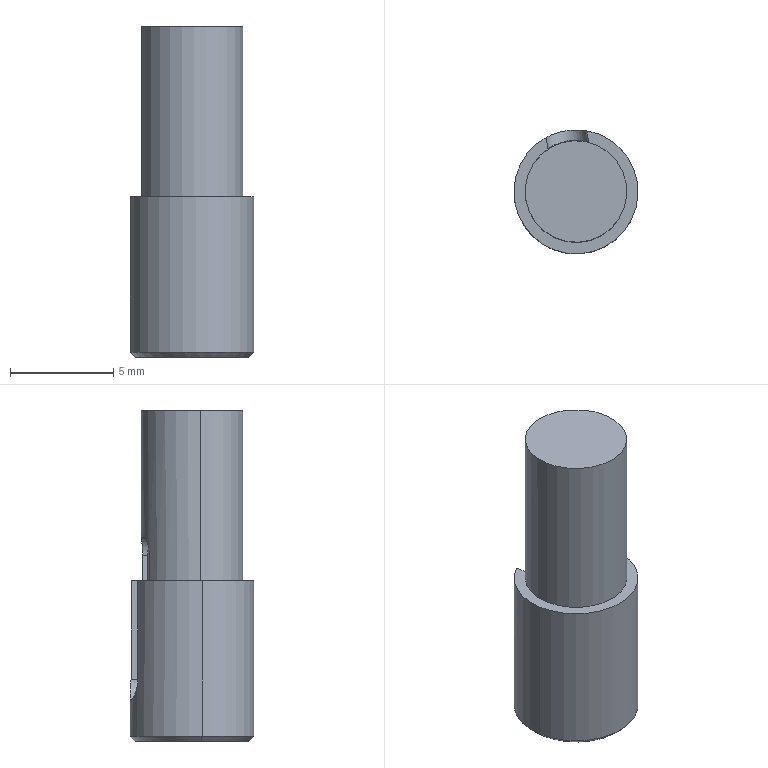Component | SolidWorks | GMotorAxis-1 | 1 solid | 18 faces | box 6 x 6 x 16 mm | volume 268 mm3 | cylinder 9 | plane 7 | cone 2 | commonest cylinder face diameters 2 x3 4.917 x2 5 x2 6 x2
STEP:
#1=COLOUR_RGB('',0.7922,0.8196,0.9333);
#2=FILL_AREA_STYLE_COLOUR('',#1);
#3=FILL_AREA_STYLE('',(#2));
#4=SURFACE_STYLE_FILL_AREA(#3);
#5=SURFACE_SIDE_STYLE('',(#4));
#6=SURFACE_STYLE_USAGE(.BOTH.,#5);
#7=PRESENTATION_STYLE_ASSIGNMENT((#6));
#8=CARTESIAN_POINT('',(-0.6803,0.01391,0.7392));
#9=VERTEX_POINT('',#8);
#10=CARTESIAN_POINT('',(-0.7226,-0.08267,0.7392));
#11=VERTEX_POINT('',#10);
#12=CARTESIAN_POINT('',(-0.6271,-0.06694,0.7392));
#13=DIRECTION('',(0.,0.,1.));
#14=DIRECTION('',(0.9867,0.1625,0.));
#15=AXIS2_PLACEMENT_3D('',#12,#13,#14);
#16=CIRCLE('',#15,0.09679);
#17=EDGE_CURVE('',#9,#11,#16,.T.);
#18=ORIENTED_EDGE('',*,*,#17,.T.);
#19=CARTESIAN_POINT('',(-0.7226,-0.08267,1.063));
#20=VERTEX_POINT('',#19);
#21=CARTESIAN_POINT('',(-0.7226,-0.08267,0.7392));
#22=DIRECTION('',(0.,0.,1.));
#23=VECTOR('',#22,39.37);
#24=LINE('',#21,#23);
#25=EDGE_CURVE('',#11,#20,#24,.T.);
#26=ORIENTED_EDGE('',*,*,#25,.T.);
#27=CARTESIAN_POINT('',(-0.5316,-0.0512,1.063));
#28=VERTEX_POINT('',#27);
#29=CARTESIAN_POINT('',(-0.6271,-0.06694,1.063));
#30=DIRECTION('',(0.,0.,1.));
#31=DIRECTION('',(0.9867,0.1625,0.));
#32=AXIS2_PLACEMENT_3D('',#29,#30,#31);
#33=CIRCLE('',#32,0.09679);
#34=EDGE_CURVE('',#28,#20,#33,.T.);
#35=ORIENTED_EDGE('',*,*,#34,.F.);
#36=CARTESIAN_POINT('',(-0.5316,-0.0512,0.7392));
#37=VERTEX_POINT('',#36);
#38=CARTESIAN_POINT('',(-0.5316,-0.0512,0.7392));
#39=DIRECTION('',(0.,0.,1.));
#40=VECTOR('',#39,39.37);
#41=LINE('',#38,#40);
#42=EDGE_CURVE('',#37,#28,#41,.T.);
#43=ORIENTED_EDGE('',*,*,#42,.F.);
#44=CARTESIAN_POINT('',(-0.6026,0.02671,0.7392));
#45=VERTEX_POINT('',#44);
#46=CARTESIAN_POINT('',(-0.6271,-0.06694,0.7392));
#47=DIRECTION('',(0.,0.,1.));
#48=DIRECTION('',(0.9867,0.1625,0.));
#49=AXIS2_PLACEMENT_3D('',#46,#47,#48);
#50=CIRCLE('',#49,0.09679);
#51=EDGE_CURVE('',#37,#45,#50,.T.);
#52=ORIENTED_EDGE('',*,*,#51,.T.);
#53=CARTESIAN_POINT('',(-0.6026,0.02671,0.7874));
#54=VERTEX_POINT('',#53);
#55=CARTESIAN_POINT('',(-0.6026,0.02671,0.7392));
#56=DIRECTION('',(0.,0.,1.));
#57=VECTOR('',#56,39.37);
#58=LINE('',#55,#57);
#59=EDGE_CURVE('',#45,#54,#58,.T.);
#60=ORIENTED_EDGE('',*,*,#59,.T.);
#61=CARTESIAN_POINT('',(-0.6428,0.02857,0.8268));
#62=VERTEX_POINT('',#61);
#63=CARTESIAN_POINT('',(-0.6026,0.02671,0.7874));
#64=CARTESIAN_POINT('',(-0.6026,0.02671,0.7927));
#65=CARTESIAN_POINT('',(-0.6037,0.02702,0.7978));
#66=CARTESIAN_POINT('',(-0.6079,0.02796,0.8073));
#67=CARTESIAN_POINT('',(-0.611,0.02858,0.8117));
#68=CARTESIAN_POINT('',(-0.6184,0.02954,0.8188));
#69=CARTESIAN_POINT('',(-0.6229,0.02988,0.8218));
#70=CARTESIAN_POINT('',(-0.6325,0.02982,0.8257));
#71=CARTESIAN_POINT('',(-0.6377,0.02941,0.8268));
#72=CARTESIAN_POINT('',(-0.6428,0.02857,0.8268));
#73=B_SPLINE_CURVE_WITH_KNOTS('',3,(#63,#64,#65,#66,#67,#68,#69,#70,#71,#72),.UNSPECIFIED.,.F.,.F.,(4,2,2,2,4),(0.,0.0003952,0.0007905,0.001186,0.001581),.UNSPECIFIED.);
#74=EDGE_CURVE('',#54,#62,#73,.T.);
#75=ORIENTED_EDGE('',*,*,#74,.T.);
#76=CARTESIAN_POINT('',(-0.6803,0.01391,0.7874));
#77=VERTEX_POINT('',#76);
#78=CARTESIAN_POINT('',(-0.6428,0.02857,0.8268));
#79=CARTESIAN_POINT('',(-0.6479,0.02772,0.8268));
#80=CARTESIAN_POINT('',(-0.653,0.02645,0.8257));
#81=CARTESIAN_POINT('',(-0.6622,0.02339,0.8217));
#82=CARTESIAN_POINT('',(-0.6663,0.02165,0.8188));
#83=CARTESIAN_POINT('',(-0.673,0.01835,0.8116));
#84=CARTESIAN_POINT('',(-0.6757,0.01679,0.8073));
#85=CARTESIAN_POINT('',(-0.6793,0.01457,0.7979));
#86=CARTESIAN_POINT('',(-0.6803,0.01391,0.7927));
#87=CARTESIAN_POINT('',(-0.6803,0.01391,0.7874));
#88=B_SPLINE_CURVE_WITH_KNOTS('',3,(#78,#79,#80,#81,#82,#83,#84,#85,#86,#87),.UNSPECIFIED.,.F.,.F.,(4,2,2,2,4),(0.001581,0.001976,0.00237,0.002765,0.003159),.UNSPECIFIED.);
#89=EDGE_CURVE('',#62,#77,#88,.T.);
#90=ORIENTED_EDGE('',*,*,#89,.T.);
#91=CARTESIAN_POINT('',(-0.6803,0.01391,0.7392));
#92=DIRECTION('',(0.,0.,-1.));
#93=VECTOR('',#92,39.37);
#94=LINE('',#91,#93);
#95=EDGE_CURVE('',#77,#9,#94,.T.);
#96=ORIENTED_EDGE('',*,*,#95,.T.);
#97=EDGE_LOOP('',(#18,#26,#35,#43,#52,#60,#75,#90,#96));
#98=FACE_OUTER_BOUND('',#97,.T.);
#99=CARTESIAN_POINT('',(-0.6271,-0.06694,0.7392));
#100=DIRECTION('',(0.,0.,1.));
#101=DIRECTION('',(0.9867,0.1625,0.));
#102=AXIS2_PLACEMENT_3D('',#99,#100,#101);
#103=CYLINDRICAL_SURFACE('',#102,0.09679);
#104=ADVANCED_FACE('',(#98),#103,.T.);
#105=CARTESIAN_POINT('',(-0.7242,-0.08293,0.6299));
#106=VERTEX_POINT('',#105);
#107=CARTESIAN_POINT('',(-0.53,-0.05094,0.6299));
#108=VERTEX_POINT('',#107);
#109=CARTESIAN_POINT('',(-0.6271,-0.06694,0.6299));
#110=DIRECTION('',(0.,0.,1.));
#111=DIRECTION('',(0.9867,0.1625,0.));
#112=AXIS2_PLACEMENT_3D('',#109,#110,#111);
#113=CIRCLE('',#112,0.09843);
#114=EDGE_CURVE('',#106,#108,#113,.T.);
#115=ORIENTED_EDGE('',*,*,#114,.T.);
#116=CARTESIAN_POINT('',(-0.53,-0.05094,0.4331));
#117=VERTEX_POINT('',#116);
#118=CARTESIAN_POINT('',(-0.53,-0.05094,0.6299));
#119=DIRECTION('',(0.,0.,-1.));
#120=VECTOR('',#119,39.37);
#121=LINE('',#118,#120);
#122=EDGE_CURVE('',#108,#117,#121,.T.);
#123=ORIENTED_EDGE('',*,*,#122,.T.);
#124=CARTESIAN_POINT('',(-0.7242,-0.08293,0.4331));
#125=VERTEX_POINT('',#124);
#126=CARTESIAN_POINT('',(-0.6271,-0.06694,0.4331));
#127=DIRECTION('',(0.,0.,-1.));
#128=DIRECTION('',(0.9867,0.1625,0.));
#129=AXIS2_PLACEMENT_3D('',#126,#127,#128);
#130=CIRCLE('',#129,0.09843);
#131=EDGE_CURVE('',#117,#125,#130,.T.);
#132=ORIENTED_EDGE('',*,*,#131,.T.);
#133=CARTESIAN_POINT('',(-0.7242,-0.08293,0.6299));
#134=DIRECTION('',(0.,0.,-1.));
#135=VECTOR('',#134,39.37);
#136=LINE('',#133,#135);
#137=EDGE_CURVE('',#106,#125,#136,.T.);
#138=ORIENTED_EDGE('',*,*,#137,.F.);
#139=EDGE_LOOP('',(#115,#123,#132,#138));
#140=FACE_OUTER_BOUND('',#139,.T.);
#141=CARTESIAN_POINT('',(-0.6271,-0.06694,0.6299));
#142=DIRECTION('',(0.,0.,-1.));
#143=DIRECTION('',(-0.9867,-0.1625,0.));
#144=AXIS2_PLACEMENT_3D('',#141,#142,#143);
#145=CYLINDRICAL_SURFACE('',#144,0.09843);
#146=ADVANCED_FACE('',(#140),#145,.F.);
#147=CARTESIAN_POINT('',(-0.7339,-0.08453,0.4331));
#148=VERTEX_POINT('',#147);
#149=CARTESIAN_POINT('',(-0.5203,-0.04934,0.4331));
#150=VERTEX_POINT('',#149);
#151=CARTESIAN_POINT('',(-0.6271,-0.06694,0.4331));
#152=DIRECTION('',(0.,0.,-1.));
#153=DIRECTION('',(0.9867,0.1625,0.));
#154=AXIS2_PLACEMENT_3D('',#151,#152,#153);
#155=CIRCLE('',#154,0.1083);
#156=EDGE_CURVE('',#148,#150,#155,.T.);
#157=ORIENTED_EDGE('',*,*,#156,.F.);
#158=CARTESIAN_POINT('',(-0.7436,-0.08613,0.4429));
#159=VERTEX_POINT('',#158);
#160=CARTESIAN_POINT('',(-0.7436,-0.08613,0.4429));
#161=DIRECTION('',(-0.6977,-0.1149,0.7071));
#162=VECTOR('',#161,39.37);
#163=LINE('',#160,#162);
#164=EDGE_CURVE('',#148,#159,#163,.T.);
#165=ORIENTED_EDGE('',*,*,#164,.T.);
#166=CARTESIAN_POINT('',(-0.5105,-0.04774,0.4429));
#167=VERTEX_POINT('',#166);
#168=CARTESIAN_POINT('',(-0.6271,-0.06694,0.4429));
#169=DIRECTION('',(0.,0.,1.));
#170=DIRECTION('',(0.9867,0.1625,0.));
#171=AXIS2_PLACEMENT_3D('',#168,#169,#170);
#172=CIRCLE('',#171,0.1181);
#173=EDGE_CURVE('',#167,#159,#172,.T.);
#174=ORIENTED_EDGE('',*,*,#173,.F.);
#175=CARTESIAN_POINT('',(-0.5105,-0.04774,0.4429));
#176=DIRECTION('',(0.6977,0.1149,0.7071));
#177=VECTOR('',#176,39.37);
#178=LINE('',#175,#177);
#179=EDGE_CURVE('',#150,#167,#178,.T.);
#180=ORIENTED_EDGE('',*,*,#179,.F.);
#181=EDGE_LOOP('',(#157,#165,#174,#180));
#182=FACE_OUTER_BOUND('',#181,.T.);
#183=CARTESIAN_POINT('',(-0.6271,-0.06694,0.4429));
#184=DIRECTION('',(0.,0.,1.));
#185=DIRECTION('',(0.9867,0.1625,0.));
#186=AXIS2_PLACEMENT_3D('',#183,#184,#185);
#187=CONICAL_SURFACE('',#186,0.1181,0.7854);
#188=ADVANCED_FACE('',(#182),#187,.T.);
#189=CARTESIAN_POINT('',(-0.5105,-0.04774,0.7392));
#190=VERTEX_POINT('',#189);
#191=CARTESIAN_POINT('',(-0.6063,0.04934,0.7392));
#192=VERTEX_POINT('',#191);
#193=CARTESIAN_POINT('',(-0.6271,-0.06694,0.7392));
#194=DIRECTION('',(0.,0.,1.));
#195=DIRECTION('',(0.9867,0.1625,0.));
#196=AXIS2_PLACEMENT_3D('',#193,#194,#195);
#197=CIRCLE('',#196,0.1181);
#198=EDGE_CURVE('',#190,#192,#197,.T.);
#199=ORIENTED_EDGE('',*,*,#198,.F.);
#200=CARTESIAN_POINT('',(-0.5105,-0.04774,1.063));
#201=DIRECTION('',(0.,0.,-1.));
#202=VECTOR('',#201,39.37);
#203=LINE('',#200,#202);
#204=EDGE_CURVE('',#190,#167,#203,.T.);
#205=ORIENTED_EDGE('',*,*,#204,.T.);
#206=ORIENTED_EDGE('',*,*,#173,.T.);
#207=CARTESIAN_POINT('',(-0.7436,-0.08613,0.7392));
#208=VERTEX_POINT('',#207);
#209=CARTESIAN_POINT('',(-0.7436,-0.08613,1.063));
#210=DIRECTION('',(0.,0.,-1.));
#211=VECTOR('',#210,39.37);
#212=LINE('',#209,#211);
#213=EDGE_CURVE('',#208,#159,#212,.T.);
#214=ORIENTED_EDGE('',*,*,#213,.F.);
#215=CARTESIAN_POINT('',(-0.684,0.03654,0.7392));
#216=VERTEX_POINT('',#215);
#217=CARTESIAN_POINT('',(-0.6271,-0.06694,0.7392));
#218=DIRECTION('',(0.,0.,1.));
#219=DIRECTION('',(0.9867,0.1625,0.));
#220=AXIS2_PLACEMENT_3D('',#217,#218,#219);
#221=CIRCLE('',#220,0.1181);
#222=EDGE_CURVE('',#216,#208,#221,.T.);
#223=ORIENTED_EDGE('',*,*,#222,.F.);
#224=CARTESIAN_POINT('',(-0.684,0.03654,0.5512));
#225=VERTEX_POINT('',#224);
#226=CARTESIAN_POINT('',(-0.684,0.03654,1.063));
#227=DIRECTION('',(0.,0.,-1.));
#228=VECTOR('',#227,39.37);
#229=LINE('',#226,#228);
#230=EDGE_CURVE('',#216,#225,#229,.T.);
#231=ORIENTED_EDGE('',*,*,#230,.T.);
#232=CARTESIAN_POINT('',(-0.6063,0.04934,0.5512));
#233=VERTEX_POINT('',#232);
#234=CARTESIAN_POINT('',(-0.6063,0.04934,0.5512));
#235=CARTESIAN_POINT('',(-0.6063,0.04934,0.5459));
#236=CARTESIAN_POINT('',(-0.6075,0.04955,0.5407));
#237=CARTESIAN_POINT('',(-0.6116,0.05017,0.5313));
#238=CARTESIAN_POINT('',(-0.6146,0.05057,0.5269));
#239=CARTESIAN_POINT('',(-0.622,0.05112,0.5197));
#240=CARTESIAN_POINT('',(-0.6264,0.05127,0.5168));
#241=CARTESIAN_POINT('',(-0.636,0.05094,0.5129));
#242=CARTESIAN_POINT('',(-0.6411,0.05045,0.5118));
#243=CARTESIAN_POINT('',(-0.6515,0.04875,0.5118));
#244=CARTESIAN_POINT('',(-0.6565,0.04755,0.5129));
#245=CARTESIAN_POINT('',(-0.6657,0.0448,0.5168));
#246=CARTESIAN_POINT('',(-0.6698,0.04324,0.5197));
#247=CARTESIAN_POINT('',(-0.6766,0.04034,0.527));
#248=CARTESIAN_POINT('',(-0.6794,0.03899,0.5313));
#249=CARTESIAN_POINT('',(-0.6831,0.03709,0.5408));
#250=CARTESIAN_POINT('',(-0.684,0.03654,0.5459));
#251=CARTESIAN_POINT('',(-0.684,0.03654,0.5512));
#252=B_SPLINE_CURVE_WITH_KNOTS('',3,(#234,#235,#236,#237,#238,#239,#240,#241,#242,#243,#244,#245,#246,#247,#248,#249,#250,#251),.UNSPECIFIED.,.F.,.F.,(4,2,2,2,2,2,2,2,4),(0.,0.000396,0.0007919,0.001188,0.001584,0.00198,0.002376,0.002772,0.003168),.UNSPECIFIED.);
#253=EDGE_CURVE('',#233,#225,#252,.T.);
#254=ORIENTED_EDGE('',*,*,#253,.F.);
#255=CARTESIAN_POINT('',(-0.6063,0.04934,1.063));
#256=DIRECTION('',(0.,0.,1.));
#257=VECTOR('',#256,39.37);
#258=LINE('',#255,#257);
#259=EDGE_CURVE('',#233,#192,#258,.T.);
#260=ORIENTED_EDGE('',*,*,#259,.T.);
#261=EDGE_LOOP('',(#199,#205,#206,#214,#223,#231,#254,#260));
#262=FACE_OUTER_BOUND('',#261,.T.);
#263=CARTESIAN_POINT('',(-0.6271,-0.06694,1.063));
#264=DIRECTION('',(0.,0.,-1.));
#265=DIRECTION('',(-0.9867,-0.1625,0.));
#266=AXIS2_PLACEMENT_3D('',#263,#264,#265);
#267=CYLINDRICAL_SURFACE('',#266,0.1181);
#268=ADVANCED_FACE('',(#262),#267,.T.);
#269=CARTESIAN_POINT('',(-0.6399,0.01076,0.8268));
#270=VERTEX_POINT('',#269);
#271=CARTESIAN_POINT('',(-0.601,0.01716,0.7874));
#272=VERTEX_POINT('',#271);
#273=CARTESIAN_POINT('',(-0.6399,0.01076,0.7874));
#274=DIRECTION('',(-0.1625,0.9867,0.));
#275=DIRECTION('',(0.,0.,-1.));
#276=AXIS2_PLACEMENT_3D('',#273,#274,#275);
#277=CIRCLE('',#276,0.03937);
#278=EDGE_CURVE('',#270,#272,#277,.T.);
#279=ORIENTED_EDGE('',*,*,#278,.F.);
#280=CARTESIAN_POINT('',(-0.6452,0.04294,0.8268));
#281=DIRECTION('',(-0.1625,0.9867,0.));
#282=VECTOR('',#281,39.37);
#283=LINE('',#280,#282);
#284=EDGE_CURVE('',#270,#62,#283,.T.);
#285=ORIENTED_EDGE('',*,*,#284,.T.);
#286=ORIENTED_EDGE('',*,*,#74,.F.);
#287=CARTESIAN_POINT('',(-0.6063,0.04934,0.7874));
#288=DIRECTION('',(-0.1625,0.9867,0.));
#289=VECTOR('',#288,39.37);
#290=LINE('',#287,#289);
#291=EDGE_CURVE('',#272,#54,#290,.T.);
#292=ORIENTED_EDGE('',*,*,#291,.F.);
#293=EDGE_LOOP('',(#279,#285,#286,#292));
#294=FACE_OUTER_BOUND('',#293,.T.);
#295=CARTESIAN_POINT('',(-0.6452,0.04294,0.7874));
#296=DIRECTION('',(-0.1625,0.9867,0.));
#297=DIRECTION('',(0.,0.,1.));
#298=AXIS2_PLACEMENT_3D('',#295,#296,#297);
#299=CYLINDRICAL_SURFACE('',#298,0.03937);
#300=ADVANCED_FACE('',(#294),#299,.F.);
#301=CARTESIAN_POINT('',(-0.6787,0.004358,0.7392));
#302=DIRECTION('',(-0.1625,0.9867,0.));
#303=VECTOR('',#302,39.37);
#304=LINE('',#301,#303);
#305=EDGE_CURVE('',#9,#216,#304,.T.);
#306=ORIENTED_EDGE('',*,*,#305,.F.);
#307=ORIENTED_EDGE('',*,*,#95,.F.);
#308=CARTESIAN_POINT('',(-0.6787,0.004358,0.7874));
#309=VERTEX_POINT('',#308);
#310=CARTESIAN_POINT('',(-0.684,0.03654,0.7874));
#311=DIRECTION('',(0.1625,-0.9867,0.));
#312=VECTOR('',#311,39.37);
#313=LINE('',#310,#312);
#314=EDGE_CURVE('',#77,#309,#313,.T.);
#315=ORIENTED_EDGE('',*,*,#314,.T.);
#316=CARTESIAN_POINT('',(-0.6787,0.004358,0.6299));
#317=VERTEX_POINT('',#316);
#318=CARTESIAN_POINT('',(-0.6787,0.004358,0.5118));
#319=DIRECTION('',(0.,0.,1.));
#320=VECTOR('',#319,39.37);
#321=LINE('',#318,#320);
#322=EDGE_CURVE('',#317,#309,#321,.T.);
#323=ORIENTED_EDGE('',*,*,#322,.F.);
#324=CARTESIAN_POINT('',(-0.6806,0.01567,0.6299));
#325=VERTEX_POINT('',#324);
#326=CARTESIAN_POINT('',(-0.6787,0.004358,0.6299));
#327=DIRECTION('',(-0.1625,0.9867,0.));
#328=VECTOR('',#327,39.37);
#329=LINE('',#326,#328);
#330=EDGE_CURVE('',#317,#325,#329,.T.);
#331=ORIENTED_EDGE('',*,*,#330,.T.);
#332=CARTESIAN_POINT('',(-0.6806,0.01567,0.5512));
#333=VERTEX_POINT('',#332);
#334=CARTESIAN_POINT('',(-0.6806,0.01567,0.6299));
#335=DIRECTION('',(0.,0.,1.));
#336=VECTOR('',#335,39.37);
#337=LINE('',#334,#336);
#338=EDGE_CURVE('',#333,#325,#337,.T.);
#339=ORIENTED_EDGE('',*,*,#338,.F.);
#340=CARTESIAN_POINT('',(-0.6787,0.004358,0.5512));
#341=DIRECTION('',(-0.1625,0.9867,0.));
#342=VECTOR('',#341,39.37);
#343=LINE('',#340,#342);
#344=EDGE_CURVE('',#333,#225,#343,.T.);
#345=ORIENTED_EDGE('',*,*,#344,.T.);
#346=ORIENTED_EDGE('',*,*,#230,.F.);
#347=EDGE_LOOP('',(#306,#307,#315,#323,#331,#339,#345,#346));
#348=FACE_OUTER_BOUND('',#347,.T.);
#349=CARTESIAN_POINT('',(-0.6787,0.004358,0.5118));
#350=DIRECTION('',(-0.9867,-0.1625,0.));
#351=DIRECTION('',(0.,0.,1.));
#352=AXIS2_PLACEMENT_3D('',#349,#350,#351);
#353=PLANE('',#352);
#354=ADVANCED_FACE('',(#348),#353,.F.);
#355=CARTESIAN_POINT('',(-0.601,0.01716,0.7392));
#356=DIRECTION('',(0.1625,-0.9867,0.));
#357=VECTOR('',#356,39.37);
#358=LINE('',#355,#357);
#359=EDGE_CURVE('',#192,#45,#358,.T.);
#360=ORIENTED_EDGE('',*,*,#359,.F.);
#361=ORIENTED_EDGE('',*,*,#259,.F.);
#362=CARTESIAN_POINT('',(-0.6029,0.02847,0.5512));
#363=VERTEX_POINT('',#362);
#364=CARTESIAN_POINT('',(-0.601,0.01716,0.5512));
#365=DIRECTION('',(0.1625,-0.9867,0.));
#366=VECTOR('',#365,39.37);
#367=LINE('',#364,#366);
#368=EDGE_CURVE('',#233,#363,#367,.T.);
#369=ORIENTED_EDGE('',*,*,#368,.T.);
#370=CARTESIAN_POINT('',(-0.6029,0.02847,0.6299));
#371=VERTEX_POINT('',#370);
#372=CARTESIAN_POINT('',(-0.6029,0.02847,0.6299));
#373=DIRECTION('',(0.,0.,-1.));
#374=VECTOR('',#373,39.37);
#375=LINE('',#372,#374);
#376=EDGE_CURVE('',#371,#363,#375,.T.);
#377=ORIENTED_EDGE('',*,*,#376,.F.);
#378=CARTESIAN_POINT('',(-0.601,0.01716,0.6299));
#379=VERTEX_POINT('',#378);
#380=CARTESIAN_POINT('',(-0.601,0.01716,0.6299));
#381=DIRECTION('',(0.1625,-0.9867,0.));
#382=VECTOR('',#381,39.37);
#383=LINE('',#380,#382);
#384=EDGE_CURVE('',#371,#379,#383,.T.);
#385=ORIENTED_EDGE('',*,*,#384,.T.);
#386=CARTESIAN_POINT('',(-0.601,0.01716,0.5118));
#387=DIRECTION('',(-0.,-0.,-1.));
#388=VECTOR('',#387,39.37);
#389=LINE('',#386,#388);
#390=EDGE_CURVE('',#272,#379,#389,.T.);
#391=ORIENTED_EDGE('',*,*,#390,.F.);
#392=ORIENTED_EDGE('',*,*,#291,.T.);
#393=ORIENTED_EDGE('',*,*,#59,.F.);
#394=EDGE_LOOP('',(#360,#361,#369,#377,#385,#391,#392,#393));
#395=FACE_OUTER_BOUND('',#394,.T.);
#396=CARTESIAN_POINT('',(-0.601,0.01716,0.5118));
#397=DIRECTION('',(0.9867,0.1625,-0.));
#398=DIRECTION('',(-0.,-0.,-1.));
#399=AXIS2_PLACEMENT_3D('',#396,#397,#398);
#400=PLANE('',#399);
#401=ADVANCED_FACE('',(#395),#400,.F.);
#402=ORIENTED_EDGE('',*,*,#284,.F.);
#403=CARTESIAN_POINT('',(-0.6399,0.01076,0.7874));
#404=DIRECTION('',(-0.1625,0.9867,0.));
#405=DIRECTION('',(0.,0.,-1.));
#406=AXIS2_PLACEMENT_3D('',#403,#404,#405);
#407=CIRCLE('',#406,0.03937);
#408=EDGE_CURVE('',#309,#270,#407,.T.);
#409=ORIENTED_EDGE('',*,*,#408,.F.);
#410=ORIENTED_EDGE('',*,*,#314,.F.);
#411=ORIENTED_EDGE('',*,*,#89,.F.);
#412=EDGE_LOOP('',(#402,#409,#410,#411));
#413=FACE_OUTER_BOUND('',#412,.T.);
#414=CARTESIAN_POINT('',(-0.6452,0.04294,0.7874));
#415=DIRECTION('',(-0.1625,0.9867,0.));
#416=DIRECTION('',(0.,0.,1.));
#417=AXIS2_PLACEMENT_3D('',#414,#415,#416);
#418=CYLINDRICAL_SURFACE('',#417,0.03937);
#419=ADVANCED_FACE('',(#413),#418,.F.);
#420=ORIENTED_EDGE('',*,*,#204,.F.);
#421=CARTESIAN_POINT('',(-0.6271,-0.06694,0.7392));
#422=DIRECTION('',(0.,0.,1.));
#423=DIRECTION('',(0.9867,0.1625,0.));
#424=AXIS2_PLACEMENT_3D('',#421,#422,#423);
#425=CIRCLE('',#424,0.1181);
#426=EDGE_CURVE('',#208,#190,#425,.T.);
#427=ORIENTED_EDGE('',*,*,#426,.F.);
#428=ORIENTED_EDGE('',*,*,#213,.T.);
#429=CARTESIAN_POINT('',(-0.6271,-0.06694,0.4429));
#430=DIRECTION('',(0.,0.,1.));
#431=DIRECTION('',(0.9867,0.1625,0.));
#432=AXIS2_PLACEMENT_3D('',#429,#430,#431);
#433=CIRCLE('',#432,0.1181);
#434=EDGE_CURVE('',#159,#167,#433,.T.);
#435=ORIENTED_EDGE('',*,*,#434,.T.);
#436=EDGE_LOOP('',(#420,#427,#428,#435));
#437=FACE_OUTER_BOUND('',#436,.T.);
#438=CARTESIAN_POINT('',(-0.6271,-0.06694,1.063));
#439=DIRECTION('',(0.,0.,-1.));
#440=DIRECTION('',(-0.9867,-0.1625,0.));
#441=AXIS2_PLACEMENT_3D('',#438,#439,#440);
#442=CYLINDRICAL_SURFACE('',#441,0.1181);
#443=ADVANCED_FACE('',(#437),#442,.T.);
#444=CARTESIAN_POINT('',(-0.6029,0.02847,0.5512));
#445=CARTESIAN_POINT('',(-0.6029,0.02847,0.5459));
#446=CARTESIAN_POINT('',(-0.604,0.02877,0.5408));
#447=CARTESIAN_POINT('',(-0.6082,0.02968,0.5313));
#448=CARTESIAN_POINT('',(-0.6112,0.03028,0.5269));
#449=CARTESIAN_POINT('',(-0.6187,0.0312,0.5198));
#450=CARTESIAN_POINT('',(-0.6231,0.03153,0.5168));
#451=CARTESIAN_POINT('',(-0.6327,0.03145,0.5129));
#452=CARTESIAN_POINT('',(-0.6379,0.03103,0.5118));
#453=CARTESIAN_POINT('',(-0.6482,0.02935,0.5118));
#454=CARTESIAN_POINT('',(-0.6532,0.02808,0.5128));
#455=CARTESIAN_POINT('',(-0.6624,0.02505,0.5168));
#456=CARTESIAN_POINT('',(-0.6665,0.02332,0.5197));
#457=CARTESIAN_POINT('',(-0.6733,0.02006,0.5269));
#458=CARTESIAN_POINT('',(-0.676,0.01851,0.5313));
#459=CARTESIAN_POINT('',(-0.6796,0.01633,0.5407));
#460=CARTESIAN_POINT('',(-0.6806,0.01567,0.5459));
#461=CARTESIAN_POINT('',(-0.6806,0.01567,0.5512));
#462=B_SPLINE_CURVE_WITH_KNOTS('',3,(#444,#445,#446,#447,#448,#449,#450,#451,#452,#453,#454,#455,#456,#457,#458,#459,#460,#461),.UNSPECIFIED.,.F.,.F.,(4,2,2,2,2,2,2,2,4),(0.,0.0003948,0.0007896,0.001184,0.001579,0.001974,0.002369,0.002764,0.003158),.UNSPECIFIED.);
#463=EDGE_CURVE('',#363,#333,#462,.T.);
#464=ORIENTED_EDGE('',*,*,#463,.F.);
#465=ORIENTED_EDGE('',*,*,#368,.F.);
#466=ORIENTED_EDGE('',*,*,#253,.T.);
#467=ORIENTED_EDGE('',*,*,#344,.F.);
#468=EDGE_LOOP('',(#464,#465,#466,#467));
#469=FACE_OUTER_BOUND('',#468,.T.);
#470=CARTESIAN_POINT('',(-0.6399,0.01076,0.5512));
#471=DIRECTION('',(-0.1625,0.9867,0.));
#472=DIRECTION('',(0.,0.,1.));
#473=AXIS2_PLACEMENT_3D('',#470,#471,#472);
#474=CYLINDRICAL_SURFACE('',#473,0.03937);
#475=ADVANCED_FACE('',(#469),#474,.F.);
#476=CARTESIAN_POINT('',(-0.6271,-0.06694,0.4331));
#477=DIRECTION('',(0.,0.,-1.));
#478=DIRECTION('',(0.9867,0.1625,0.));
#479=AXIS2_PLACEMENT_3D('',#476,#477,#478);
#480=CIRCLE('',#479,0.09843);
#481=EDGE_CURVE('',#125,#117,#480,.T.);
#482=ORIENTED_EDGE('',*,*,#481,.F.);
#483=ORIENTED_EDGE('',*,*,#131,.F.);
#484=EDGE_LOOP('',(#482,#483));
#485=FACE_BOUND('',#484,.T.);
#486=CARTESIAN_POINT('',(-0.6271,-0.06694,0.4331));
#487=DIRECTION('',(0.,0.,-1.));
#488=DIRECTION('',(0.9867,0.1625,0.));
#489=AXIS2_PLACEMENT_3D('',#486,#487,#488);
#490=CIRCLE('',#489,0.1083);
#491=EDGE_CURVE('',#150,#148,#490,.T.);
#492=ORIENTED_EDGE('',*,*,#491,.T.);
#493=ORIENTED_EDGE('',*,*,#156,.T.);
#494=EDGE_LOOP('',(#492,#493));
#495=FACE_OUTER_BOUND('',#494,.T.);
#496=CARTESIAN_POINT('',(-0.6271,-0.06694,0.4331));
#497=DIRECTION('',(0.,0.,1.));
#498=DIRECTION('',(0.9867,0.1625,0.));
#499=AXIS2_PLACEMENT_3D('',#496,#497,#498);
#500=PLANE('',#499);
#501=ADVANCED_FACE('',(#485,#495),#500,.F.);
#502=ORIENTED_EDGE('',*,*,#390,.T.);
#503=CARTESIAN_POINT('',(-0.6399,0.01076,0.6299));
#504=DIRECTION('',(-0.9867,-0.1625,0.));
#505=VECTOR('',#504,39.37);
#506=LINE('',#503,#505);
#507=EDGE_CURVE('',#379,#317,#506,.T.);
#508=ORIENTED_EDGE('',*,*,#507,.T.);
#509=ORIENTED_EDGE('',*,*,#322,.T.);
#510=ORIENTED_EDGE('',*,*,#408,.T.);
#511=ORIENTED_EDGE('',*,*,#278,.T.);
#512=EDGE_LOOP('',(#502,#508,#509,#510,#511));
#513=FACE_OUTER_BOUND('',#512,.T.);
#514=CARTESIAN_POINT('',(-0.6399,0.01076,0.4331));
#515=DIRECTION('',(0.1625,-0.9867,0.));
#516=DIRECTION('',(0.,0.,-1.));
#517=AXIS2_PLACEMENT_3D('',#514,#515,#516);
#518=PLANE('',#517);
#519=ADVANCED_FACE('',(#513),#518,.F.);
#520=ORIENTED_EDGE('',*,*,#164,.F.);
#521=ORIENTED_EDGE('',*,*,#491,.F.);
#522=ORIENTED_EDGE('',*,*,#179,.T.);
#523=ORIENTED_EDGE('',*,*,#434,.F.);
#524=EDGE_LOOP('',(#520,#521,#522,#523));
#525=FACE_OUTER_BOUND('',#524,.T.);
#526=CARTESIAN_POINT('',(-0.6271,-0.06694,0.4429));
#527=DIRECTION('',(0.,0.,1.));
#528=DIRECTION('',(0.9867,0.1625,0.));
#529=AXIS2_PLACEMENT_3D('',#526,#527,#528);
#530=CONICAL_SURFACE('',#529,0.1181,0.7854);
#531=ADVANCED_FACE('',(#525),#530,.T.);
#532=ORIENTED_EDGE('',*,*,#122,.F.);
#533=CARTESIAN_POINT('',(-0.6271,-0.06694,0.6299));
#534=DIRECTION('',(0.,0.,1.));
#535=DIRECTION('',(0.9867,0.1625,0.));
#536=AXIS2_PLACEMENT_3D('',#533,#534,#535);
#537=CIRCLE('',#536,0.09843);
#538=EDGE_CURVE('',#108,#371,#537,.T.);
#539=ORIENTED_EDGE('',*,*,#538,.T.);
#540=ORIENTED_EDGE('',*,*,#376,.T.);
#541=ORIENTED_EDGE('',*,*,#463,.T.);
#542=ORIENTED_EDGE('',*,*,#338,.T.);
#543=CARTESIAN_POINT('',(-0.6271,-0.06694,0.6299));
#544=DIRECTION('',(0.,0.,1.));
#545=DIRECTION('',(0.9867,0.1625,0.));
#546=AXIS2_PLACEMENT_3D('',#543,#544,#545);
#547=CIRCLE('',#546,0.09843);
#548=EDGE_CURVE('',#325,#106,#547,.T.);
#549=ORIENTED_EDGE('',*,*,#548,.T.);
#550=ORIENTED_EDGE('',*,*,#137,.T.);
#551=ORIENTED_EDGE('',*,*,#481,.T.);
#552=EDGE_LOOP('',(#532,#539,#540,#541,#542,#549,#550,#551));
#553=FACE_OUTER_BOUND('',#552,.T.);
#554=CARTESIAN_POINT('',(-0.6271,-0.06694,0.6299));
#555=DIRECTION('',(0.,0.,-1.));
#556=DIRECTION('',(-0.9867,-0.1625,0.));
#557=AXIS2_PLACEMENT_3D('',#554,#555,#556);
#558=CYLINDRICAL_SURFACE('',#557,0.09843);
#559=ADVANCED_FACE('',(#553),#558,.F.);
#560=ORIENTED_EDGE('',*,*,#507,.F.);
#561=ORIENTED_EDGE('',*,*,#384,.F.);
#562=ORIENTED_EDGE('',*,*,#538,.F.);
#563=ORIENTED_EDGE('',*,*,#114,.F.);
#564=ORIENTED_EDGE('',*,*,#548,.F.);
#565=ORIENTED_EDGE('',*,*,#330,.F.);
#566=EDGE_LOOP('',(#560,#561,#562,#563,#564,#565));
#567=FACE_OUTER_BOUND('',#566,.T.);
#568=CARTESIAN_POINT('',(-0.6271,-0.06694,0.6299));
#569=DIRECTION('',(0.,0.,1.));
#570=DIRECTION('',(0.9867,0.1625,0.));
#571=AXIS2_PLACEMENT_3D('',#568,#569,#570);
#572=PLANE('',#571);
#573=ADVANCED_FACE('',(#567),#572,.F.);
#574=ORIENTED_EDGE('',*,*,#305,.T.);
#575=ORIENTED_EDGE('',*,*,#222,.T.);
#576=ORIENTED_EDGE('',*,*,#426,.T.);
#577=ORIENTED_EDGE('',*,*,#198,.T.);
#578=ORIENTED_EDGE('',*,*,#359,.T.);
#579=ORIENTED_EDGE('',*,*,#51,.F.);
#580=CARTESIAN_POINT('',(-0.6271,-0.06694,0.7392));
#581=DIRECTION('',(0.,0.,1.));
#582=DIRECTION('',(0.9867,0.1625,0.));
#583=AXIS2_PLACEMENT_3D('',#580,#581,#582);
#584=CIRCLE('',#583,0.09679);
#585=EDGE_CURVE('',#11,#37,#584,.T.);
#586=ORIENTED_EDGE('',*,*,#585,.F.);
#587=ORIENTED_EDGE('',*,*,#17,.F.);
#588=EDGE_LOOP('',(#574,#575,#576,#577,#578,#579,#586,#587));
#589=FACE_OUTER_BOUND('',#588,.T.);
#590=CARTESIAN_POINT('',(-0.6271,-0.06694,0.7392));
#591=DIRECTION('',(0.,0.,1.));
#592=DIRECTION('',(0.9867,0.1625,0.));
#593=AXIS2_PLACEMENT_3D('',#590,#591,#592);
#594=PLANE('',#593);
#595=ADVANCED_FACE('',(#589),#594,.T.);
#596=ORIENTED_EDGE('',*,*,#25,.F.);
#597=ORIENTED_EDGE('',*,*,#585,.T.);
#598=ORIENTED_EDGE('',*,*,#42,.T.);
#599=CARTESIAN_POINT('',(-0.6271,-0.06694,1.063));
#600=DIRECTION('',(0.,0.,1.));
#601=DIRECTION('',(0.9867,0.1625,0.));
#602=AXIS2_PLACEMENT_3D('',#599,#600,#601);
#603=CIRCLE('',#602,0.09679);
#604=EDGE_CURVE('',#20,#28,#603,.T.);
#605=ORIENTED_EDGE('',*,*,#604,.F.);
#606=EDGE_LOOP('',(#596,#597,#598,#605));
#607=FACE_OUTER_BOUND('',#606,.T.);
#608=CARTESIAN_POINT('',(-0.6271,-0.06694,0.7392));
#609=DIRECTION('',(0.,0.,1.));
#610=DIRECTION('',(0.9867,0.1625,0.));
#611=AXIS2_PLACEMENT_3D('',#608,#609,#610);
#612=CYLINDRICAL_SURFACE('',#611,0.09679);
#613=ADVANCED_FACE('',(#607),#612,.T.);
#614=ORIENTED_EDGE('',*,*,#34,.T.);
#615=ORIENTED_EDGE('',*,*,#604,.T.);
#616=EDGE_LOOP('',(#614,#615));
#617=FACE_OUTER_BOUND('',#616,.T.);
#618=CARTESIAN_POINT('',(-0.6271,-0.06694,1.063));
#619=DIRECTION('',(0.,0.,1.));
#620=DIRECTION('',(0.9867,0.1625,0.));
#621=AXIS2_PLACEMENT_3D('',#618,#619,#620);
#622=PLANE('',#621);
#623=ADVANCED_FACE('',(#617),#622,.T.);
#624=CLOSED_SHELL('',(#104,#146,#188,#268,#300,#354,#401,#419,#443,#475,#501,#519,#531,#559,#573,#595,#613,#623));
#625=MANIFOLD_SOLID_BREP('',#624);
#626=STYLED_ITEM('',(#7),#625);
#627=PRESENTATION_LAYER_ASSIGNMENT('','',(#626));
#628=CARTESIAN_POINT('',(0.,0.,0.));
#629=DIRECTION('',(0.,0.,1.));
#630=DIRECTION('',(1.,0.,0.));
#631=AXIS2_PLACEMENT_3D('',#628,#629,#630);
#632=(LENGTH_UNIT()NAMED_UNIT(*)SI_UNIT($,.METRE.));
#633=LENGTH_MEASURE_WITH_UNIT(LENGTH_MEASURE(0.0254),#632);
#634=DIMENSIONAL_EXPONENTS(1.,0.,0.,0.,0.,0.,0.);
#635=(CONVERSION_BASED_UNIT('',#633)LENGTH_UNIT()NAMED_UNIT(#634));
#636=UNCERTAINTY_MEASURE_WITH_UNIT(LENGTH_MEASURE(0.00001),#635,'','');
#637=(NAMED_UNIT(*)PLANE_ANGLE_UNIT()SI_UNIT($,.RADIAN.));
#638=(NAMED_UNIT(*)SI_UNIT($,.STERADIAN.)SOLID_ANGLE_UNIT());
#639=(GEOMETRIC_REPRESENTATION_CONTEXT(3)GLOBAL_UNCERTAINTY_ASSIGNED_CONTEXT((#636))GLOBAL_UNIT_ASSIGNED_CONTEXT((#635,#637,#638))REPRESENTATION_CONTEXT('',''));
#640=ADVANCED_BREP_SHAPE_REPRESENTATION('',(#625,#631),#639);
#641=(LENGTH_UNIT()NAMED_UNIT(*)SI_UNIT($,.METRE.));
#642=LENGTH_MEASURE_WITH_UNIT(LENGTH_MEASURE(0.0254),#641);
#643=DIMENSIONAL_EXPONENTS(1.,0.,0.,0.,0.,0.,0.);
#644=(CONVERSION_BASED_UNIT('',#642)LENGTH_UNIT()NAMED_UNIT(#643));
#645=UNCERTAINTY_MEASURE_WITH_UNIT(LENGTH_MEASURE(0.00001),#644,'','');
#646=(NAMED_UNIT(*)PLANE_ANGLE_UNIT()SI_UNIT($,.RADIAN.));
#647=(NAMED_UNIT(*)SI_UNIT($,.STERADIAN.)SOLID_ANGLE_UNIT());
#648=(GEOMETRIC_REPRESENTATION_CONTEXT(3)GLOBAL_UNCERTAINTY_ASSIGNED_CONTEXT((#645))GLOBAL_UNIT_ASSIGNED_CONTEXT((#644,#646,#647))REPRESENTATION_CONTEXT('',''));
#649=MECHANICAL_DESIGN_GEOMETRIC_PRESENTATION_REPRESENTATION('',(#626),#648);